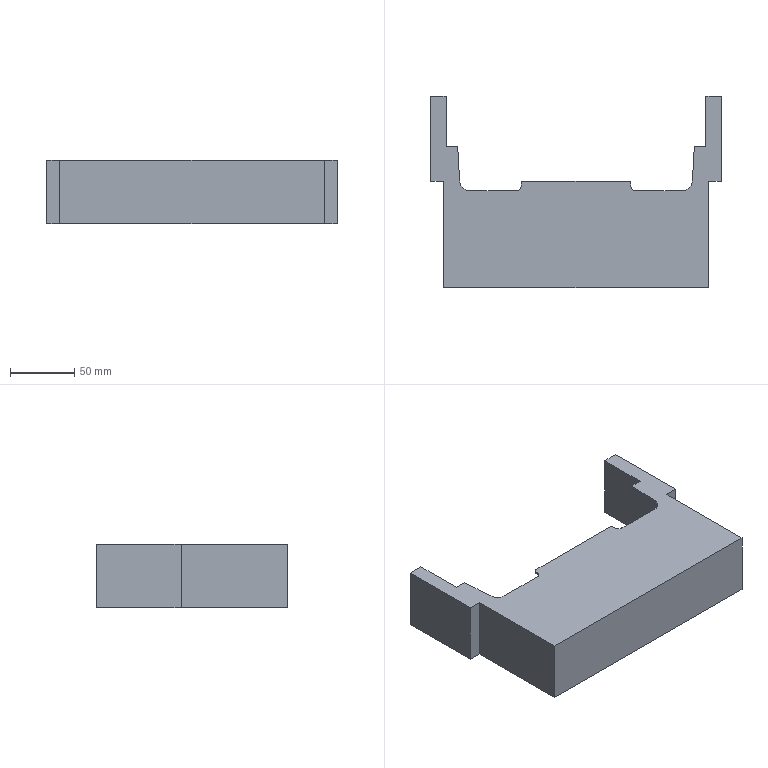Component | NX | HOPPER | 1 solid | 30 faces | volume 146086 mm3 | plane 24 | cylinder 6 | commonest cylinder face diameters 16 x2 8 x2 4 x2